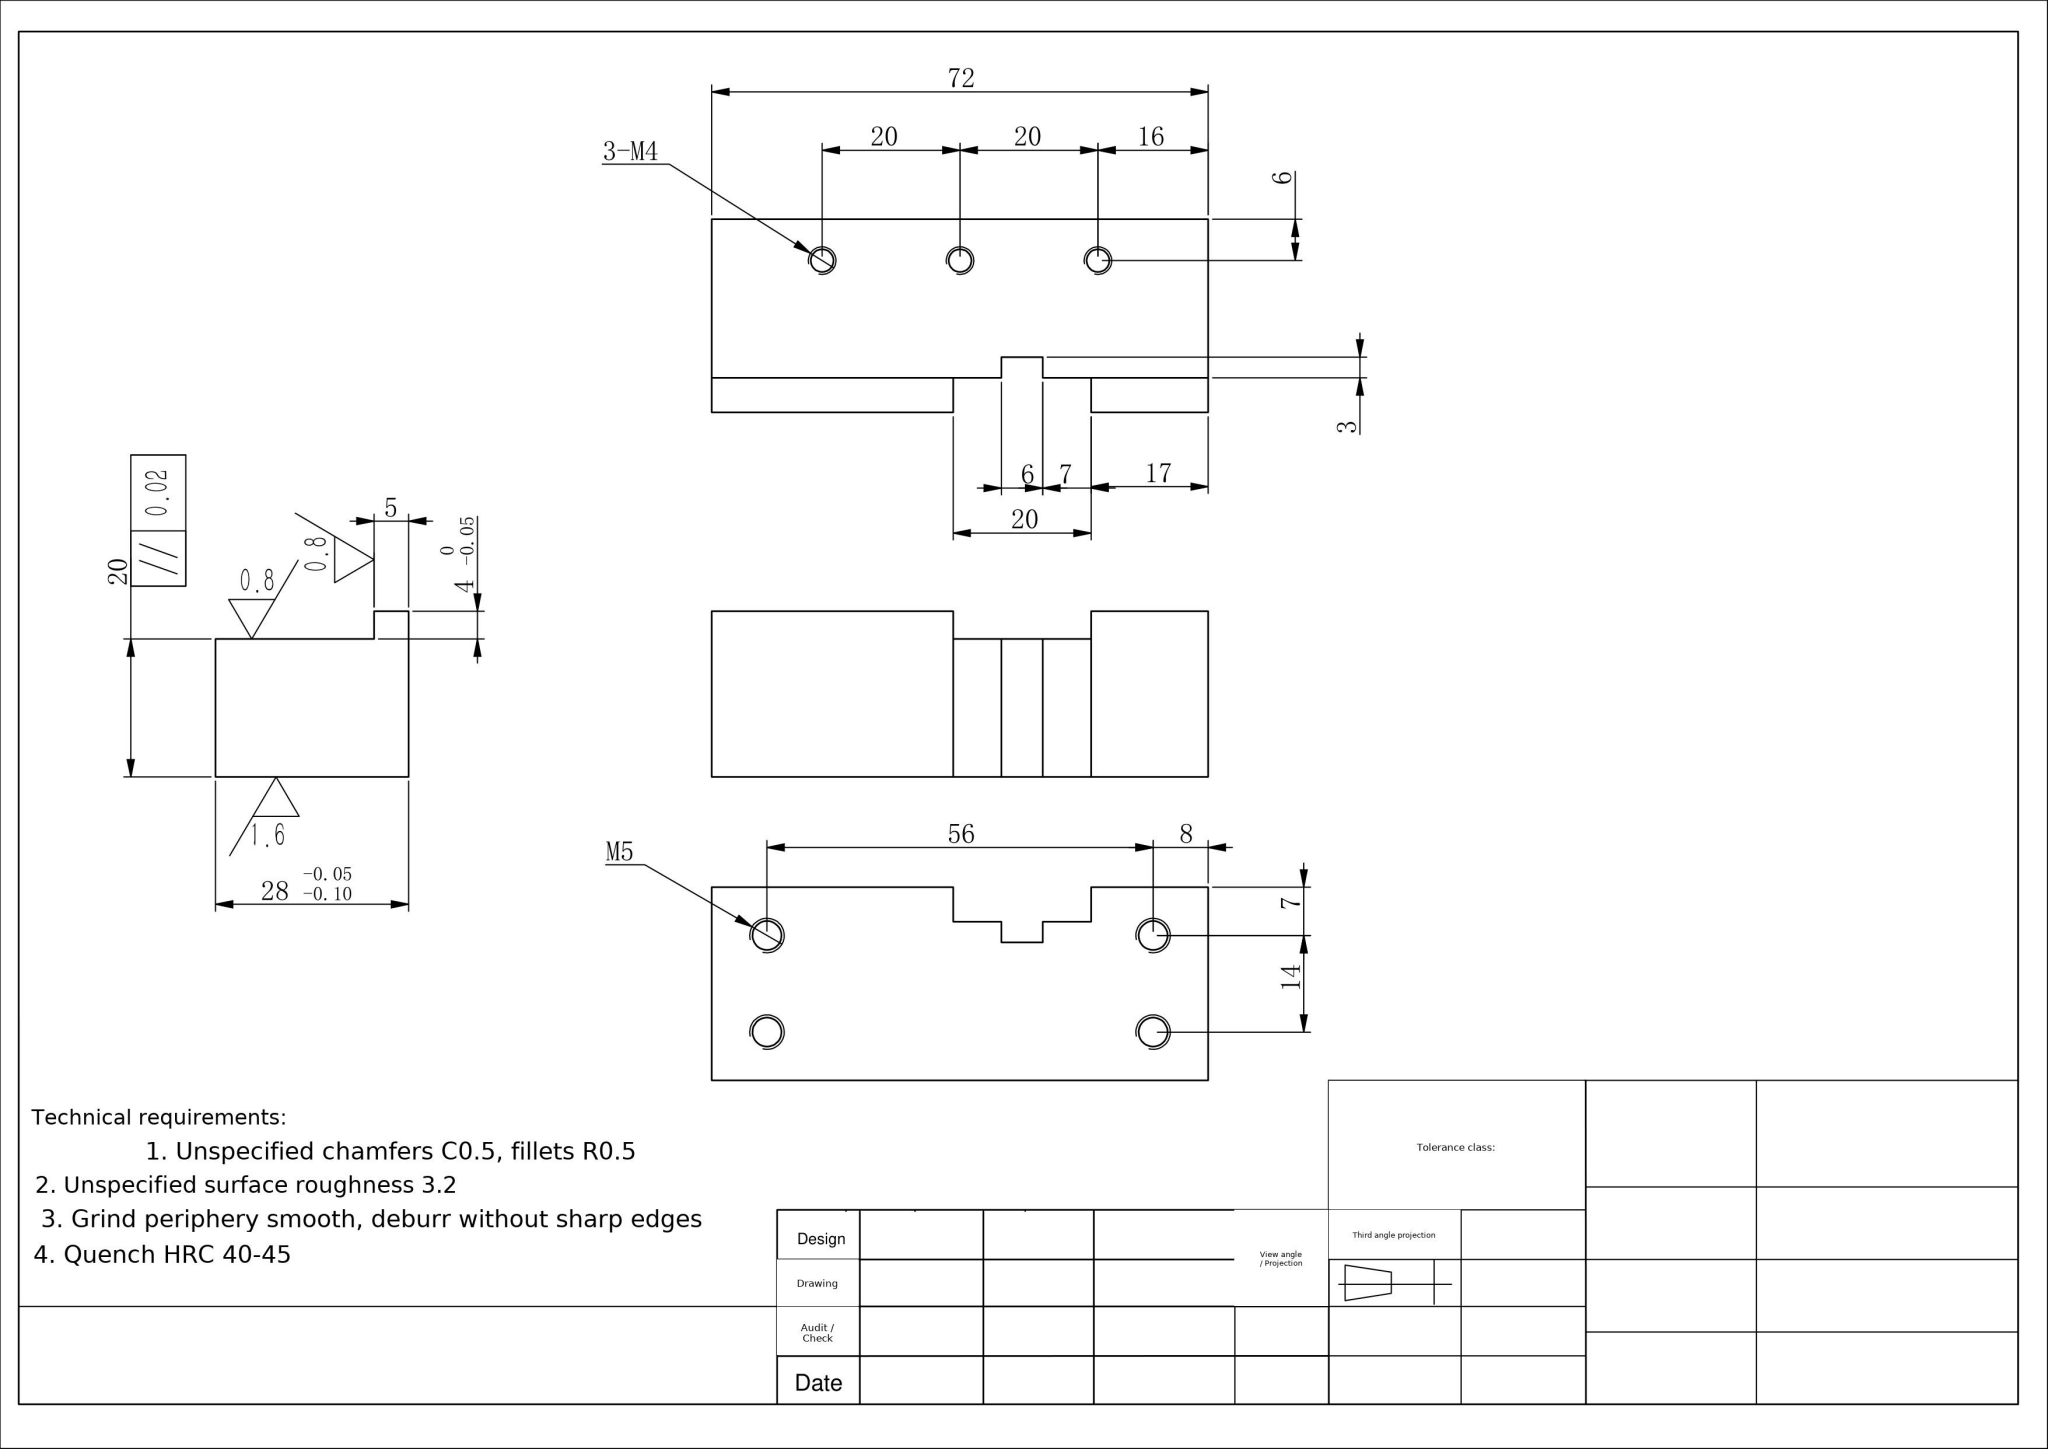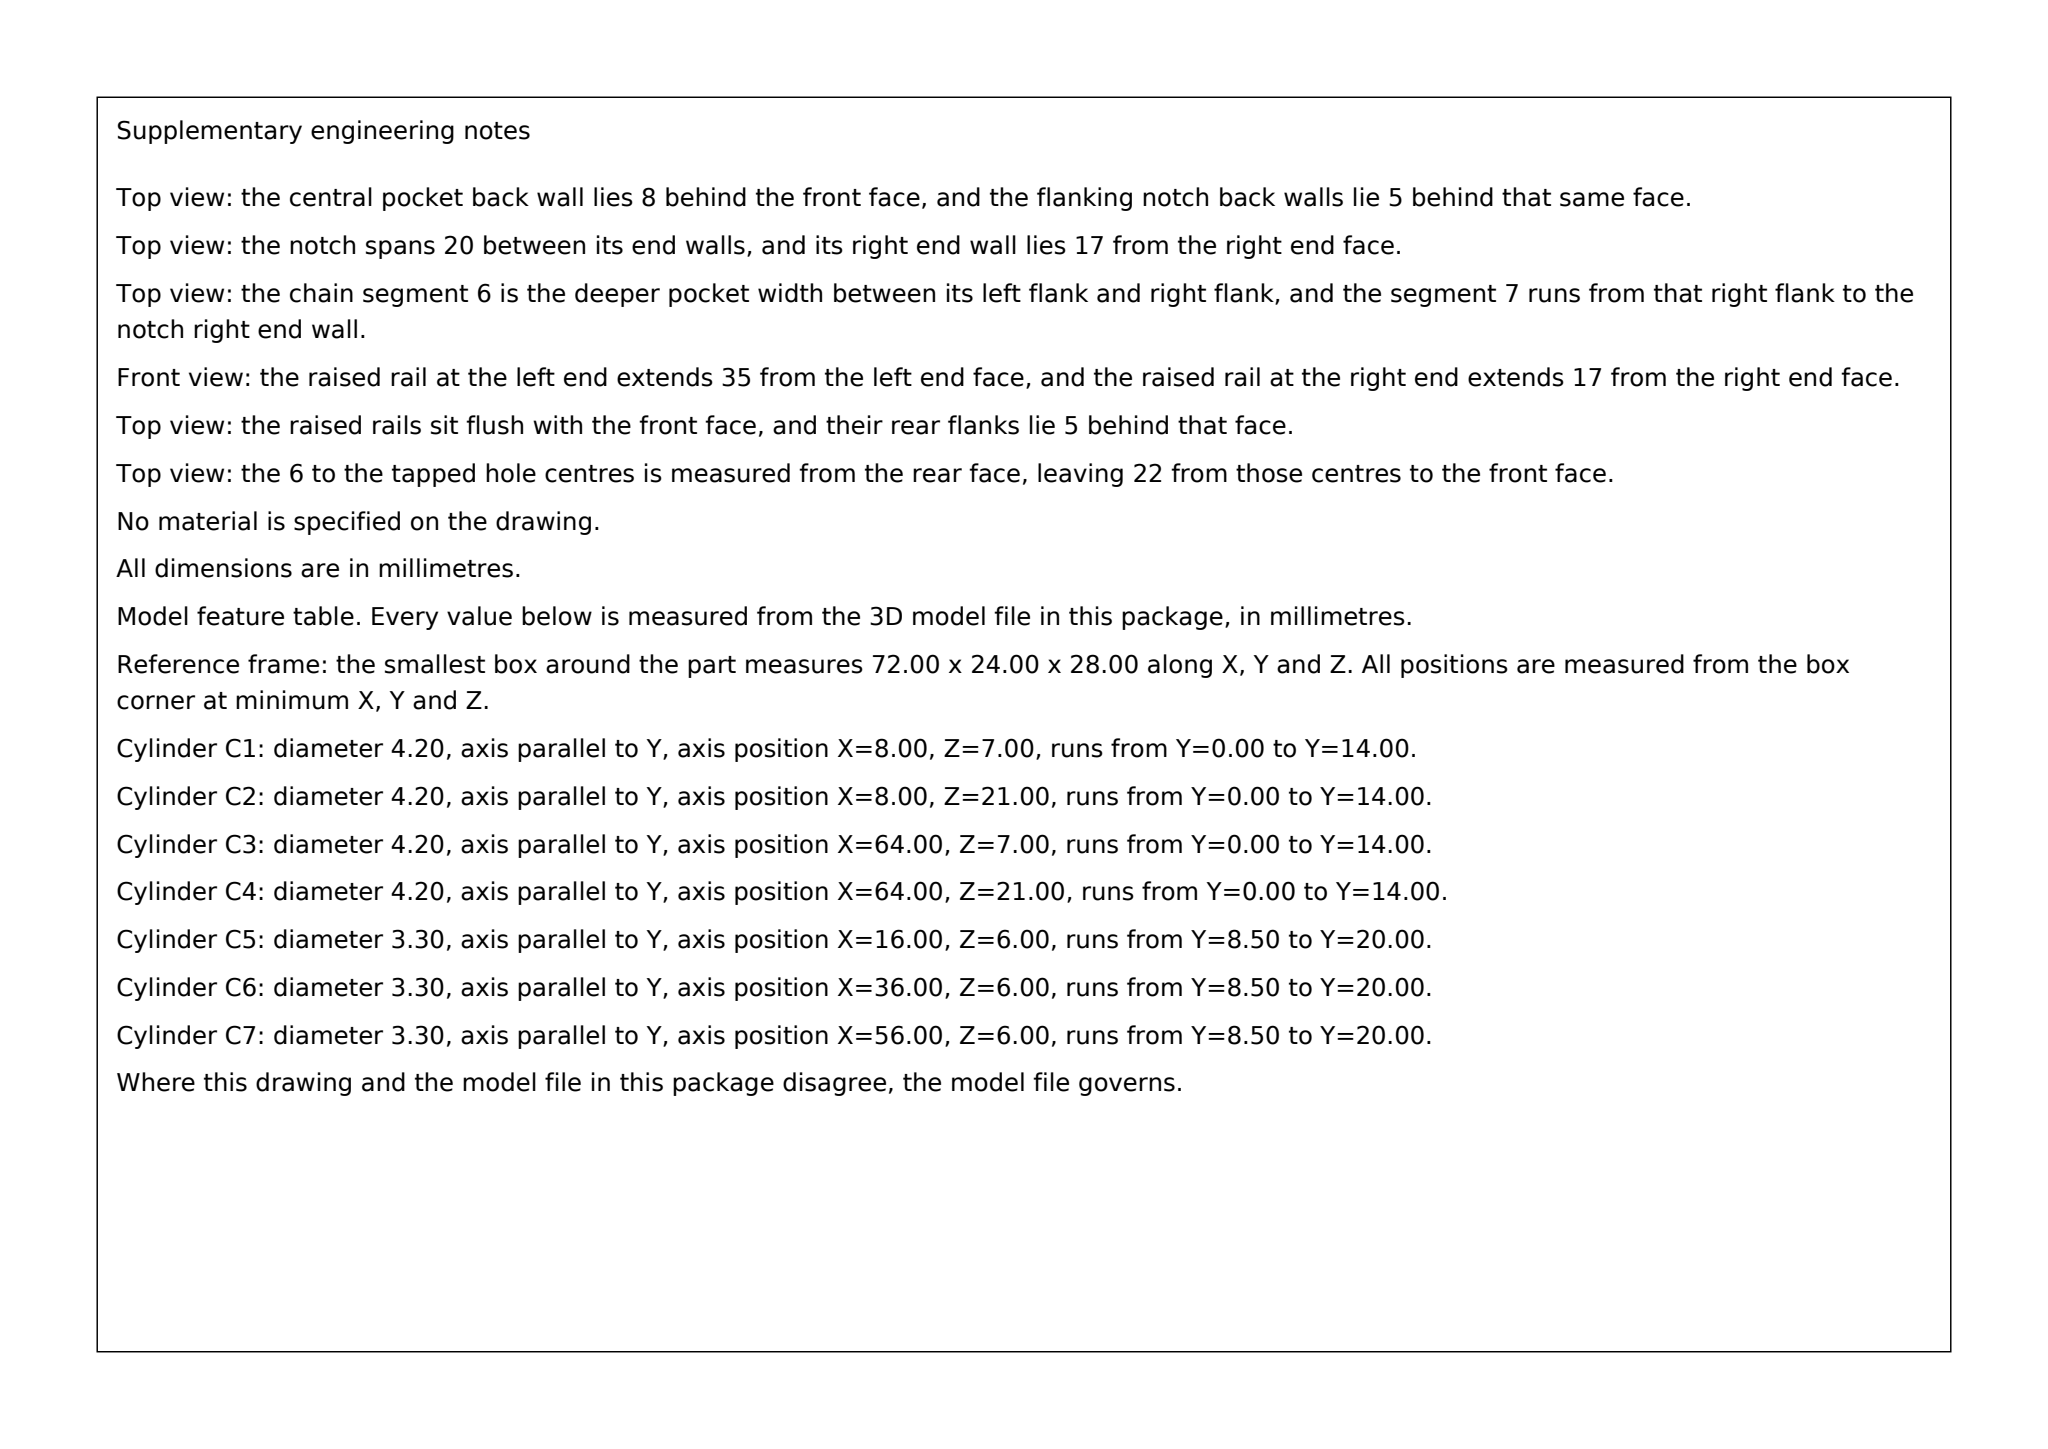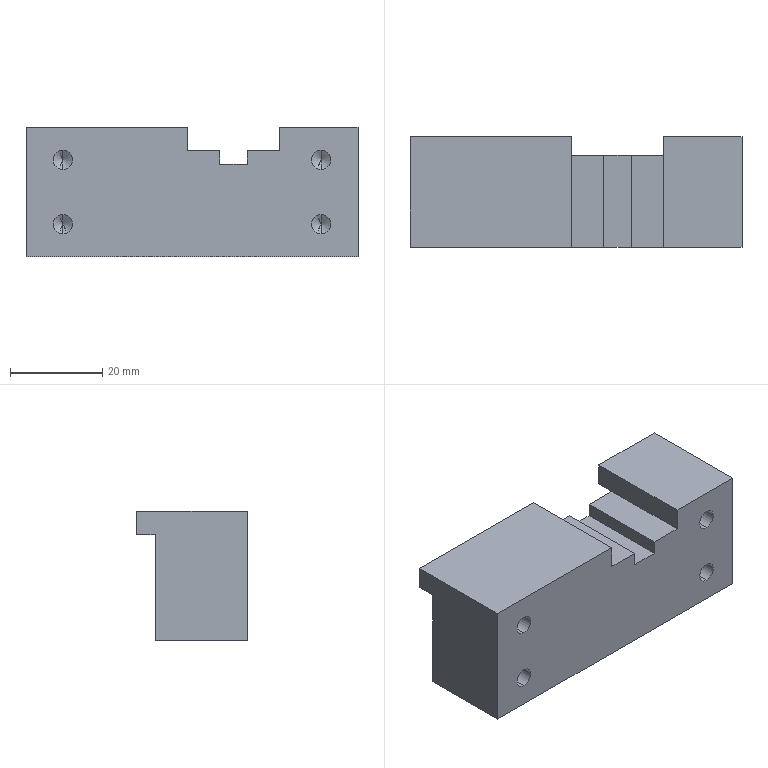Part | SolidWorks | mm | 1 solid | 46 faces | box 72 x 24 x 28 mm | volume 37897 mm3 | plane 18 | cylinder 14 | cone 14 | commonest cylinder face diameters 4.2 x8 3.3 x6
Drawing notes:
UPPER VIEW: 3-M4 DP 11.5, EQ SP 20, 6 FROM TOP EDGE | from the solid: 3x ø3.3 y-axis holes, L=11.5, at x=16/36/56, z=6; 118° drill point
LOWER VIEW: 4-M5 DP 14, 56 APART x 14 APART, 8 & 7 FROM EDGES | from the solid: 4x ø4.2 y-axis holes, L=14, at x=8/64, z=7/21; 118° drill point
build123d program:
from build123d import *

# Parameters (mm, degrees)
SKETCH1_W             = 28
SKETCH1_H             = 24
BOSS_EXTRUDE1_DEPTH   = 72
SKETCH2_W             = 23
SKETCH2_H             = 4
CUT_EXTRUDE1_DEPTH    = 81.895
SKETCH4_W             = 20
SKETCH4_H             = 5
CUT_EXTRUDE3_DEPTH    = 81.895
SKETCH15_W            = 6
SKETCH15_H            = 3
CUT_EXTRUDE4_DEPTH    = 80.8
M5_TAPPED_HOLE1_D     = 4.2
M5_TAPPED_HOLE1_DEPTH = 14
M5_TAPPED_HOLE1_TIP   = 1.262
M4_TAPPED_HOLE2_D     = 3.3
M4_TAPPED_HOLE2_DEPTH = 11.5
M4_TAPPED_HOLE2_TIP   = 0.9914


with BuildPart() as part:
    # Sketch1 → Boss-Extrude1 (new body)
    with BuildSketch(Plane(origin=(0, 0, 0), x_dir=(0, 0, -1), z_dir=(1, 0, 0))):
        with Locations((14, 12)):
            Rectangle(SKETCH1_W, SKETCH1_H)
    extrude(amount=BOSS_EXTRUDE1_DEPTH)

    # Sketch2 → Cut-Extrude1 (cut, through all)
    with BuildSketch(Plane(origin=(72, 0, 0), x_dir=(0, 0, -1), z_dir=(1, 0, 0))):
        with Locations((16.5, 22)):
            Rectangle(SKETCH2_W, SKETCH2_H)
    extrude(amount=-CUT_EXTRUDE1_DEPTH, mode=Mode.SUBTRACT)

    # Sketch4 → Cut-Extrude3 (cut, through all)
    with BuildSketch(Plane(origin=(0, 24, 0), x_dir=(1, 0, 0), z_dir=(0, 1, 0))):
        with Locations((45, 2.5)):
            Rectangle(SKETCH4_W, SKETCH4_H)
    extrude(amount=-CUT_EXTRUDE3_DEPTH, mode=Mode.SUBTRACT)

    # Sketch15 → Cut-Extrude4 (cut, through all)
    with BuildSketch(Plane(origin=(0, 20, 0), x_dir=(1, 0, 0), z_dir=(0, 1, 0))):
        with Locations((45, 6.5)):
            Rectangle(SKETCH15_W, SKETCH15_H)
    extrude(amount=-CUT_EXTRUDE4_DEPTH, mode=Mode.SUBTRACT)

    # M5 Tapped Hole1
    with Locations(Plane(origin=(0, 0, 0), x_dir=(-1, 0, 0), z_dir=(0, -1, 0))):
        with Locations((-8, 7), (-8, 21), (-64, 21), (-64, 7)):
            Hole(M5_TAPPED_HOLE1_D / 2, depth=M5_TAPPED_HOLE1_DEPTH)
            with Locations((0, 0, -(M5_TAPPED_HOLE1_DEPTH + M5_TAPPED_HOLE1_TIP / 2))):  # 118° drill point
                Cone(0, M5_TAPPED_HOLE1_D / 2, M5_TAPPED_HOLE1_TIP, mode=Mode.SUBTRACT)

    # M4 Tapped Hole2
    with Locations(Plane(origin=(0, 20, 0), x_dir=(1, 0, 0), z_dir=(0, 1, 0))):
        with Locations((56, 22), (36, 22), (16, 22)):
            Hole(M4_TAPPED_HOLE2_D / 2, depth=M4_TAPPED_HOLE2_DEPTH)
            with Locations((0, 0, -(M4_TAPPED_HOLE2_DEPTH + M4_TAPPED_HOLE2_TIP / 2))):  # 118° drill point
                Cone(0, M4_TAPPED_HOLE2_D / 2, M4_TAPPED_HOLE2_TIP, mode=Mode.SUBTRACT)


solid = part.part